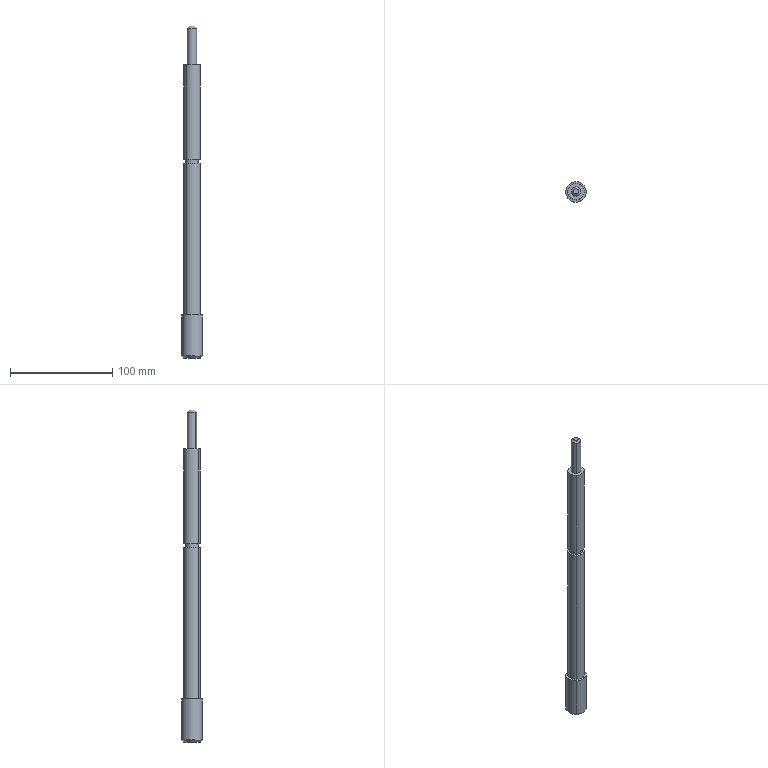Component | SolidWorks | 12-1 | 1 solid | 26 faces | box 20 x 20 x 324 mm | volume 64045 mm3 | cylinder 13 | plane 9 | cone 4 | commonest cylinder face diameters 16 x4 5 x3 9 x2 12 x2 20 x2
build123d program:
from build123d import *

# Parameters (mm, degrees)
CHAMFER1_SIZE      = 2
CUT_EXTRUDE1_START = -8
CUT_EXTRUDE1_DEPTH = 1.8


with BuildPart() as part:
    # Sketch1 → Revolve1 (revolve)
    with BuildSketch(Plane.XY, mode=Mode.PRIVATE) as revolve1_sk:
        Polygon((0, 0), (0, 10), (42, 10), (42, 8), (190, 8), (190, 6), (194, 6), (194, 8), (286, 8), (286, 4.5), (324, 4.5), (324, 0), align=None)
    revolve(revolve1_sk.sketch.rotate(Axis((324, 0, 0), (-1, 0, 0)), 90), axis=Axis((324, 0, 0), (-1, 0, 0)))

    # Chamfer1
    chamfer1_edges = [part.edges().sort_by_distance(p)[0] for p in [
        (0, 0, 10),
        (324, 0, 4.5),
    ]]
    chamfer(chamfer1_edges, length=CHAMFER1_SIZE)

    # Sketch2 → Cut-Extrude1 (cut)
    with BuildSketch(Plane.XY.offset(CUT_EXTRUDE1_START)):
        with BuildLine():
            Line((107, 2.5), (116, 2.5))
            ThreePointArc((116, 2.5), (118.5, 0), (116, -2.5))
            Line((116, -2.5), (107, -2.5))
            ThreePointArc((107, -2.5), (104.5, 0), (107, 2.5))
        make_face()
    extrude(amount=CUT_EXTRUDE1_DEPTH, mode=Mode.SUBTRACT)


solid = part.part

# Placed as in the assembly
solid = solid.moved(Location((-135.043, 380.991, 493.213), (90, -40.335, 90)))
STEP:
#1=COLOUR_RGB('',0.7922,0.8196,0.9333);
#2=FILL_AREA_STYLE_COLOUR('',#1);
#3=FILL_AREA_STYLE('',(#2));
#4=SURFACE_STYLE_FILL_AREA(#3);
#5=SURFACE_SIDE_STYLE('',(#4));
#6=SURFACE_STYLE_USAGE(.BOTH.,#5);
#7=PRESENTATION_STYLE_ASSIGNMENT((#6));
#8=CARTESIAN_POINT('',(-5.234,15.249,23.63));
#9=VERTEX_POINT('',#8);
#10=CARTESIAN_POINT('',(-5.159,15.186,23.532));
#11=VERTEX_POINT('',#10);
#12=CARTESIAN_POINT('',(-5.159,15.186,23.63));
#13=DIRECTION('',(-0.6473,-0.7623,0.));
#14=DIRECTION('',(0.,0.,1.));
#15=AXIS2_PLACEMENT_3D('',#12,#13,#14);
#16=CIRCLE('',#15,0.09843);
#17=EDGE_CURVE('',#9,#11,#16,.T.);
#18=ORIENTED_EDGE('',*,*,#17,.T.);
#19=CARTESIAN_POINT('',(-5.113,15.24,23.532));
#20=VERTEX_POINT('',#19);
#21=CARTESIAN_POINT('',(-5.159,15.186,23.532));
#22=DIRECTION('',(0.6473,0.7623,-0.));
#23=VECTOR('',#22,39.37);
#24=LINE('',#21,#23);
#25=EDGE_CURVE('',#11,#20,#24,.T.);
#26=ORIENTED_EDGE('',*,*,#25,.T.);
#27=CARTESIAN_POINT('',(-5.198,15.291,23.63));
#28=VERTEX_POINT('',#27);
#29=CARTESIAN_POINT('',(-5.198,15.291,23.63));
#30=CARTESIAN_POINT('',(-5.198,15.291,23.624));
#31=CARTESIAN_POINT('',(-5.197,15.291,23.617));
#32=CARTESIAN_POINT('',(-5.195,15.29,23.605));
#33=CARTESIAN_POINT('',(-5.193,15.289,23.599));
#34=CARTESIAN_POINT('',(-5.188,15.287,23.587));
#35=CARTESIAN_POINT('',(-5.185,15.286,23.581));
#36=CARTESIAN_POINT('',(-5.179,15.283,23.57));
#37=CARTESIAN_POINT('',(-5.175,15.281,23.565));
#38=CARTESIAN_POINT('',(-5.163,15.275,23.552));
#39=CARTESIAN_POINT('',(-5.153,15.269,23.544));
#40=CARTESIAN_POINT('',(-5.138,15.259,23.537));
#41=CARTESIAN_POINT('',(-5.133,15.256,23.535));
#42=CARTESIAN_POINT('',(-5.123,15.248,23.533));
#43=CARTESIAN_POINT('',(-5.118,15.244,23.532));
#44=CARTESIAN_POINT('',(-5.113,15.24,23.532));
#45=B_SPLINE_CURVE_WITH_KNOTS('',3,(#29,#30,#31,#32,#33,#34,#35,#36,#37,#38,#39,#40,#41,#42,#43,#44),.UNSPECIFIED.,.F.,.F.,(4,2,2,2,2,2,2,4),(0.,0.0004917,0.0009835,0.001475,0.001967,0.00295,0.003442,0.003934),.UNSPECIFIED.);
#46=EDGE_CURVE('',#28,#20,#45,.T.);
#47=ORIENTED_EDGE('',*,*,#46,.F.);
#48=CARTESIAN_POINT('',(-5.234,15.249,23.63));
#49=DIRECTION('',(0.6473,0.7623,-0.));
#50=VECTOR('',#49,39.37);
#51=LINE('',#48,#50);
#52=EDGE_CURVE('',#9,#28,#51,.T.);
#53=ORIENTED_EDGE('',*,*,#52,.F.);
#54=EDGE_LOOP('',(#18,#26,#47,#53));
#55=FACE_OUTER_BOUND('',#54,.T.);
#56=CARTESIAN_POINT('',(-5.159,15.186,23.63));
#57=DIRECTION('',(0.6473,0.7623,-0.));
#58=DIRECTION('',(0.,0.,-1.));
#59=AXIS2_PLACEMENT_3D('',#56,#57,#58);
#60=CYLINDRICAL_SURFACE('',#59,0.09843);
#61=ADVANCED_FACE('',(#55),#60,.F.);
#62=CARTESIAN_POINT('',(-5.521,14.76,19.418));
#63=VERTEX_POINT('',#62);
#64=CARTESIAN_POINT('',(-5.113,15.24,19.418));
#65=VERTEX_POINT('',#64);
#66=CARTESIAN_POINT('',(-5.317,15.,19.418));
#67=DIRECTION('',(-0.,-0.,-1.));
#68=DIRECTION('',(-0.6473,-0.7623,0.));
#69=AXIS2_PLACEMENT_3D('',#66,#67,#68);
#70=CIRCLE('',#69,0.315);
#71=EDGE_CURVE('',#63,#65,#70,.T.);
#72=ORIENTED_EDGE('',*,*,#71,.F.);
#73=CARTESIAN_POINT('',(-5.571,14.7,19.497));
#74=VERTEX_POINT('',#73);
#75=CARTESIAN_POINT('',(-5.571,14.7,19.497));
#76=DIRECTION('',(-0.4577,-0.539,0.7071));
#77=VECTOR('',#76,39.37);
#78=LINE('',#75,#77);
#79=EDGE_CURVE('',#63,#74,#78,.T.);
#80=ORIENTED_EDGE('',*,*,#79,.T.);
#81=CARTESIAN_POINT('',(-5.062,15.3,19.497));
#82=VERTEX_POINT('',#81);
#83=CARTESIAN_POINT('',(-5.317,15.,19.497));
#84=DIRECTION('',(0.,0.,1.));
#85=DIRECTION('',(-0.6473,-0.7623,0.));
#86=AXIS2_PLACEMENT_3D('',#83,#84,#85);
#87=CIRCLE('',#86,0.3937);
#88=EDGE_CURVE('',#82,#74,#87,.T.);
#89=ORIENTED_EDGE('',*,*,#88,.F.);
#90=CARTESIAN_POINT('',(-5.062,15.3,19.497));
#91=DIRECTION('',(0.4577,0.539,0.7071));
#92=VECTOR('',#91,39.37);
#93=LINE('',#90,#92);
#94=EDGE_CURVE('',#65,#82,#93,.T.);
#95=ORIENTED_EDGE('',*,*,#94,.F.);
#96=EDGE_LOOP('',(#72,#80,#89,#95));
#97=FACE_OUTER_BOUND('',#96,.T.);
#98=CARTESIAN_POINT('',(-5.317,15.,19.497));
#99=DIRECTION('',(0.,0.,1.));
#100=DIRECTION('',(0.6473,0.7623,0.));
#101=AXIS2_PLACEMENT_3D('',#98,#99,#100);
#102=CONICAL_SURFACE('',#101,0.3937,0.7854);
#103=ADVANCED_FACE('',(#97),#102,.T.);
#104=CARTESIAN_POINT('',(-5.253,15.075,32.174));
#105=VERTEX_POINT('',#104);
#106=CARTESIAN_POINT('',(-5.38,14.925,32.174));
#107=VERTEX_POINT('',#106);
#108=CARTESIAN_POINT('',(-5.317,15.,32.174));
#109=DIRECTION('',(0.,0.,1.));
#110=DIRECTION('',(0.6473,0.7623,0.));
#111=AXIS2_PLACEMENT_3D('',#108,#109,#110);
#112=CIRCLE('',#111,0.09843);
#113=EDGE_CURVE('',#105,#107,#112,.T.);
#114=ORIENTED_EDGE('',*,*,#113,.F.);
#115=CARTESIAN_POINT('',(-5.202,15.135,32.095));
#116=VERTEX_POINT('',#115);
#117=CARTESIAN_POINT('',(-5.253,15.075,32.174));
#118=DIRECTION('',(0.4577,0.539,-0.7071));
#119=VECTOR('',#118,39.37);
#120=LINE('',#117,#119);
#121=EDGE_CURVE('',#105,#116,#120,.T.);
#122=ORIENTED_EDGE('',*,*,#121,.T.);
#123=CARTESIAN_POINT('',(-5.431,14.865,32.095));
#124=VERTEX_POINT('',#123);
#125=CARTESIAN_POINT('',(-5.317,15.,32.095));
#126=DIRECTION('',(-0.,-0.,-1.));
#127=DIRECTION('',(0.6473,0.7623,0.));
#128=AXIS2_PLACEMENT_3D('',#125,#126,#127);
#129=CIRCLE('',#128,0.1772);
#130=EDGE_CURVE('',#124,#116,#129,.T.);
#131=ORIENTED_EDGE('',*,*,#130,.F.);
#132=CARTESIAN_POINT('',(-5.38,14.925,32.174));
#133=DIRECTION('',(-0.4577,-0.539,-0.7071));
#134=VECTOR('',#133,39.37);
#135=LINE('',#132,#134);
#136=EDGE_CURVE('',#107,#124,#135,.T.);
#137=ORIENTED_EDGE('',*,*,#136,.F.);
#138=EDGE_LOOP('',(#114,#122,#131,#137));
#139=FACE_OUTER_BOUND('',#138,.T.);
#140=CARTESIAN_POINT('',(-5.317,15.,32.174));
#141=DIRECTION('',(-0.,-0.,-1.));
#142=DIRECTION('',(-0.6473,-0.7623,0.));
#143=AXIS2_PLACEMENT_3D('',#140,#141,#142);
#144=CONICAL_SURFACE('',#143,0.09843,0.7854);
#145=ADVANCED_FACE('',(#139),#144,.T.);
#146=CARTESIAN_POINT('',(-5.202,15.135,30.678));
#147=VERTEX_POINT('',#146);
#148=CARTESIAN_POINT('',(-5.431,14.865,30.678));
#149=VERTEX_POINT('',#148);
#150=CARTESIAN_POINT('',(-5.317,15.,30.678));
#151=DIRECTION('',(0.,0.,1.));
#152=DIRECTION('',(0.6473,0.7623,0.));
#153=AXIS2_PLACEMENT_3D('',#150,#151,#152);
#154=CIRCLE('',#153,0.1772);
#155=EDGE_CURVE('',#147,#149,#154,.T.);
#156=ORIENTED_EDGE('',*,*,#155,.T.);
#157=CARTESIAN_POINT('',(-5.431,14.865,32.174));
#158=DIRECTION('',(0.,0.,1.));
#159=VECTOR('',#158,39.37);
#160=LINE('',#157,#159);
#161=EDGE_CURVE('',#149,#124,#160,.T.);
#162=ORIENTED_EDGE('',*,*,#161,.T.);
#163=ORIENTED_EDGE('',*,*,#130,.T.);
#164=CARTESIAN_POINT('',(-5.202,15.135,32.174));
#165=DIRECTION('',(0.,0.,1.));
#166=VECTOR('',#165,39.37);
#167=LINE('',#164,#166);
#168=EDGE_CURVE('',#147,#116,#167,.T.);
#169=ORIENTED_EDGE('',*,*,#168,.F.);
#170=EDGE_LOOP('',(#156,#162,#163,#169));
#171=FACE_OUTER_BOUND('',#170,.T.);
#172=CARTESIAN_POINT('',(-5.317,15.,32.174));
#173=DIRECTION('',(0.,0.,1.));
#174=DIRECTION('',(0.6473,0.7623,0.));
#175=AXIS2_PLACEMENT_3D('',#172,#173,#174);
#176=CYLINDRICAL_SURFACE('',#175,0.1772);
#177=ADVANCED_FACE('',(#171),#176,.T.);
#178=CARTESIAN_POINT('',(-5.113,15.24,27.056));
#179=VERTEX_POINT('',#178);
#180=CARTESIAN_POINT('',(-5.521,14.76,27.056));
#181=VERTEX_POINT('',#180);
#182=CARTESIAN_POINT('',(-5.317,15.,27.056));
#183=DIRECTION('',(0.,0.,1.));
#184=DIRECTION('',(0.6473,0.7623,0.));
#185=AXIS2_PLACEMENT_3D('',#182,#183,#184);
#186=CIRCLE('',#185,0.315);
#187=EDGE_CURVE('',#179,#181,#186,.T.);
#188=ORIENTED_EDGE('',*,*,#187,.T.);
#189=CARTESIAN_POINT('',(-5.521,14.76,30.678));
#190=VERTEX_POINT('',#189);
#191=CARTESIAN_POINT('',(-5.521,14.76,32.174));
#192=DIRECTION('',(0.,0.,1.));
#193=VECTOR('',#192,39.37);
#194=LINE('',#191,#193);
#195=EDGE_CURVE('',#181,#190,#194,.T.);
#196=ORIENTED_EDGE('',*,*,#195,.T.);
#197=CARTESIAN_POINT('',(-5.113,15.24,30.678));
#198=VERTEX_POINT('',#197);
#199=CARTESIAN_POINT('',(-5.317,15.,30.678));
#200=DIRECTION('',(0.,0.,1.));
#201=DIRECTION('',(0.6473,0.7623,0.));
#202=AXIS2_PLACEMENT_3D('',#199,#200,#201);
#203=CIRCLE('',#202,0.315);
#204=EDGE_CURVE('',#198,#190,#203,.T.);
#205=ORIENTED_EDGE('',*,*,#204,.F.);
#206=CARTESIAN_POINT('',(-5.113,15.24,32.174));
#207=DIRECTION('',(0.,0.,1.));
#208=VECTOR('',#207,39.37);
#209=LINE('',#206,#208);
#210=EDGE_CURVE('',#179,#198,#209,.T.);
#211=ORIENTED_EDGE('',*,*,#210,.F.);
#212=EDGE_LOOP('',(#188,#196,#205,#211));
#213=FACE_OUTER_BOUND('',#212,.T.);
#214=CARTESIAN_POINT('',(-5.317,15.,32.174));
#215=DIRECTION('',(0.,0.,1.));
#216=DIRECTION('',(0.6473,0.7623,0.));
#217=AXIS2_PLACEMENT_3D('',#214,#215,#216);
#218=CYLINDRICAL_SURFACE('',#217,0.315);
#219=ADVANCED_FACE('',(#213),#218,.T.);
#220=CARTESIAN_POINT('',(-5.164,15.18,26.898));
#221=VERTEX_POINT('',#220);
#222=CARTESIAN_POINT('',(-5.47,14.82,26.898));
#223=VERTEX_POINT('',#222);
#224=CARTESIAN_POINT('',(-5.317,15.,26.898));
#225=DIRECTION('',(0.,0.,1.));
#226=DIRECTION('',(0.6473,0.7623,0.));
#227=AXIS2_PLACEMENT_3D('',#224,#225,#226);
#228=CIRCLE('',#227,0.2362);
#229=EDGE_CURVE('',#221,#223,#228,.T.);
#230=ORIENTED_EDGE('',*,*,#229,.T.);
#231=CARTESIAN_POINT('',(-5.47,14.82,27.056));
#232=VERTEX_POINT('',#231);
#233=CARTESIAN_POINT('',(-5.47,14.82,32.174));
#234=DIRECTION('',(0.,0.,1.));
#235=VECTOR('',#234,39.37);
#236=LINE('',#233,#235);
#237=EDGE_CURVE('',#223,#232,#236,.T.);
#238=ORIENTED_EDGE('',*,*,#237,.T.);
#239=CARTESIAN_POINT('',(-5.164,15.18,27.056));
#240=VERTEX_POINT('',#239);
#241=CARTESIAN_POINT('',(-5.317,15.,27.056));
#242=DIRECTION('',(0.,0.,1.));
#243=DIRECTION('',(0.6473,0.7623,0.));
#244=AXIS2_PLACEMENT_3D('',#241,#242,#243);
#245=CIRCLE('',#244,0.2362);
#246=EDGE_CURVE('',#240,#232,#245,.T.);
#247=ORIENTED_EDGE('',*,*,#246,.F.);
#248=CARTESIAN_POINT('',(-5.164,15.18,32.174));
#249=DIRECTION('',(0.,0.,1.));
#250=VECTOR('',#249,39.37);
#251=LINE('',#248,#250);
#252=EDGE_CURVE('',#221,#240,#251,.T.);
#253=ORIENTED_EDGE('',*,*,#252,.F.);
#254=EDGE_LOOP('',(#230,#238,#247,#253));
#255=FACE_OUTER_BOUND('',#254,.T.);
#256=CARTESIAN_POINT('',(-5.317,15.,32.174));
#257=DIRECTION('',(0.,0.,1.));
#258=DIRECTION('',(0.6473,0.7623,0.));
#259=AXIS2_PLACEMENT_3D('',#256,#257,#258);
#260=CYLINDRICAL_SURFACE('',#259,0.2362);
#261=ADVANCED_FACE('',(#255),#260,.T.);
#262=ORIENTED_EDGE('',*,*,#88,.T.);
#263=CARTESIAN_POINT('',(-5.571,14.7,21.071));
#264=VERTEX_POINT('',#263);
#265=CARTESIAN_POINT('',(-5.571,14.7,32.174));
#266=DIRECTION('',(0.,0.,1.));
#267=VECTOR('',#266,39.37);
#268=LINE('',#265,#267);
#269=EDGE_CURVE('',#74,#264,#268,.T.);
#270=ORIENTED_EDGE('',*,*,#269,.T.);
#271=CARTESIAN_POINT('',(-5.062,15.3,21.071));
#272=VERTEX_POINT('',#271);
#273=CARTESIAN_POINT('',(-5.317,15.,21.071));
#274=DIRECTION('',(0.,0.,1.));
#275=DIRECTION('',(0.6473,0.7623,0.));
#276=AXIS2_PLACEMENT_3D('',#273,#274,#275);
#277=CIRCLE('',#276,0.3937);
#278=EDGE_CURVE('',#272,#264,#277,.T.);
#279=ORIENTED_EDGE('',*,*,#278,.F.);
#280=CARTESIAN_POINT('',(-5.062,15.3,32.174));
#281=DIRECTION('',(0.,0.,1.));
#282=VECTOR('',#281,39.37);
#283=LINE('',#280,#282);
#284=EDGE_CURVE('',#82,#272,#283,.T.);
#285=ORIENTED_EDGE('',*,*,#284,.F.);
#286=EDGE_LOOP('',(#262,#270,#279,#285));
#287=FACE_OUTER_BOUND('',#286,.T.);
#288=CARTESIAN_POINT('',(-5.317,15.,32.174));
#289=DIRECTION('',(0.,0.,1.));
#290=DIRECTION('',(0.6473,0.7623,0.));
#291=AXIS2_PLACEMENT_3D('',#288,#289,#290);
#292=CYLINDRICAL_SURFACE('',#291,0.3937);
#293=ADVANCED_FACE('',(#287),#292,.T.);
#294=CARTESIAN_POINT('',(-5.113,15.24,21.071));
#295=VERTEX_POINT('',#294);
#296=CARTESIAN_POINT('',(-5.521,14.76,21.071));
#297=VERTEX_POINT('',#296);
#298=CARTESIAN_POINT('',(-5.317,15.,21.071));
#299=DIRECTION('',(0.,0.,1.));
#300=DIRECTION('',(0.6473,0.7623,0.));
#301=AXIS2_PLACEMENT_3D('',#298,#299,#300);
#302=CIRCLE('',#301,0.315);
#303=EDGE_CURVE('',#295,#297,#302,.T.);
#304=ORIENTED_EDGE('',*,*,#303,.T.);
#305=CARTESIAN_POINT('',(-5.521,14.76,26.898));
#306=VERTEX_POINT('',#305);
#307=CARTESIAN_POINT('',(-5.521,14.76,32.174));
#308=DIRECTION('',(0.,0.,1.));
#309=VECTOR('',#308,39.37);
#310=LINE('',#307,#309);
#311=EDGE_CURVE('',#297,#306,#310,.T.);
#312=ORIENTED_EDGE('',*,*,#311,.T.);
#313=CARTESIAN_POINT('',(-5.113,15.24,26.898));
#314=VERTEX_POINT('',#313);
#315=CARTESIAN_POINT('',(-5.317,15.,26.898));
#316=DIRECTION('',(0.,0.,1.));
#317=DIRECTION('',(0.6473,0.7623,0.));
#318=AXIS2_PLACEMENT_3D('',#315,#316,#317);
#319=CIRCLE('',#318,0.315);
#320=EDGE_CURVE('',#314,#306,#319,.T.);
#321=ORIENTED_EDGE('',*,*,#320,.F.);
#322=CARTESIAN_POINT('',(-5.113,15.24,24.083));
#323=VERTEX_POINT('',#322);
#324=CARTESIAN_POINT('',(-5.113,15.24,32.174));
#325=DIRECTION('',(0.,0.,1.));
#326=VECTOR('',#325,39.37);
#327=LINE('',#324,#326);
#328=EDGE_CURVE('',#323,#314,#327,.T.);
#329=ORIENTED_EDGE('',*,*,#328,.F.);
#330=CARTESIAN_POINT('',(-5.198,15.291,23.985));
#331=VERTEX_POINT('',#330);
#332=CARTESIAN_POINT('',(-5.113,15.24,24.083));
#333=CARTESIAN_POINT('',(-5.118,15.244,24.083));
#334=CARTESIAN_POINT('',(-5.123,15.248,24.083));
#335=CARTESIAN_POINT('',(-5.133,15.256,24.08));
#336=CARTESIAN_POINT('',(-5.138,15.259,24.078));
#337=CARTESIAN_POINT('',(-5.148,15.266,24.073));
#338=CARTESIAN_POINT('',(-5.153,15.269,24.07));
#339=CARTESIAN_POINT('',(-5.162,15.274,24.063));
#340=CARTESIAN_POINT('',(-5.167,15.277,24.059));
#341=CARTESIAN_POINT('',(-5.175,15.281,24.05));
#342=CARTESIAN_POINT('',(-5.179,15.283,24.045));
#343=CARTESIAN_POINT('',(-5.185,15.286,24.034));
#344=CARTESIAN_POINT('',(-5.188,15.287,24.029));
#345=CARTESIAN_POINT('',(-5.193,15.289,24.017));
#346=CARTESIAN_POINT('',(-5.195,15.29,24.011));
#347=CARTESIAN_POINT('',(-5.197,15.291,23.998));
#348=CARTESIAN_POINT('',(-5.198,15.291,23.991));
#349=CARTESIAN_POINT('',(-5.198,15.291,23.985));
#350=B_SPLINE_CURVE_WITH_KNOTS('',3,(#332,#333,#334,#335,#336,#337,#338,#339,#340,#341,#342,#343,#344,#345,#346,#347,#348,#349),.UNSPECIFIED.,.F.,.F.,(4,2,2,2,2,2,2,2,4),(0.003934,0.004425,0.004916,0.005407,0.005898,0.006389,0.006881,0.007372,0.007863),.UNSPECIFIED.);
#351=EDGE_CURVE('',#323,#331,#350,.T.);
#352=ORIENTED_EDGE('',*,*,#351,.T.);
#353=CARTESIAN_POINT('',(-5.198,15.291,32.174));
#354=DIRECTION('',(-0.,-0.,-1.));
#355=VECTOR('',#354,39.37);
#356=LINE('',#353,#355);
#357=EDGE_CURVE('',#331,#28,#356,.T.);
#358=ORIENTED_EDGE('',*,*,#357,.T.);
#359=ORIENTED_EDGE('',*,*,#46,.T.);
#360=CARTESIAN_POINT('',(-5.113,15.24,32.174));
#361=DIRECTION('',(0.,0.,1.));
#362=VECTOR('',#361,39.37);
#363=LINE('',#360,#362);
#364=EDGE_CURVE('',#295,#20,#363,.T.);
#365=ORIENTED_EDGE('',*,*,#364,.F.);
#366=EDGE_LOOP('',(#304,#312,#321,#329,#352,#358,#359,#365));
#367=FACE_OUTER_BOUND('',#366,.T.);
#368=CARTESIAN_POINT('',(-5.317,15.,32.174));
#369=DIRECTION('',(0.,0.,1.));
#370=DIRECTION('',(0.6473,0.7623,0.));
#371=AXIS2_PLACEMENT_3D('',#368,#369,#370);
#372=CYLINDRICAL_SURFACE('',#371,0.315);
#373=ADVANCED_FACE('',(#367),#372,.T.);
#374=ORIENTED_EDGE('',*,*,#311,.F.);
#375=CARTESIAN_POINT('',(-5.317,15.,21.071));
#376=DIRECTION('',(0.,0.,1.));
#377=DIRECTION('',(0.6473,0.7623,0.));
#378=AXIS2_PLACEMENT_3D('',#375,#376,#377);
#379=CIRCLE('',#378,0.315);
#380=EDGE_CURVE('',#297,#295,#379,.T.);
#381=ORIENTED_EDGE('',*,*,#380,.T.);
#382=ORIENTED_EDGE('',*,*,#364,.T.);
#383=CARTESIAN_POINT('',(-5.048,15.164,23.63));
#384=VERTEX_POINT('',#383);
#385=CARTESIAN_POINT('',(-5.113,15.24,23.532));
#386=CARTESIAN_POINT('',(-5.108,15.236,23.532));
#387=CARTESIAN_POINT('',(-5.103,15.231,23.533));
#388=CARTESIAN_POINT('',(-5.094,15.222,23.535));
#389=CARTESIAN_POINT('',(-5.09,15.218,23.537));
#390=CARTESIAN_POINT('',(-5.081,15.209,23.542));
#391=CARTESIAN_POINT('',(-5.078,15.205,23.545));
#392=CARTESIAN_POINT('',(-5.071,15.196,23.552));
#393=CARTESIAN_POINT('',(-5.068,15.192,23.556));
#394=CARTESIAN_POINT('',(-5.062,15.185,23.565));
#395=CARTESIAN_POINT('',(-5.06,15.182,23.57));
#396=CARTESIAN_POINT('',(-5.055,15.176,23.581));
#397=CARTESIAN_POINT('',(-5.054,15.173,23.587));
#398=CARTESIAN_POINT('',(-5.051,15.169,23.599));
#399=CARTESIAN_POINT('',(-5.05,15.167,23.605));
#400=CARTESIAN_POINT('',(-5.048,15.165,23.617));
#401=CARTESIAN_POINT('',(-5.048,15.164,23.624));
#402=CARTESIAN_POINT('',(-5.048,15.164,23.63));
#403=B_SPLINE_CURVE_WITH_KNOTS('',3,(#385,#386,#387,#388,#389,#390,#391,#392,#393,#394,#395,#396,#397,#398,#399,#400,#401,#402),.UNSPECIFIED.,.F.,.F.,(4,2,2,2,2,2,2,2,4),(0.003934,0.004425,0.004916,0.005407,0.005898,0.006389,0.006881,0.007372,0.007863),.UNSPECIFIED.);
#404=EDGE_CURVE('',#20,#384,#403,.T.);
#405=ORIENTED_EDGE('',*,*,#404,.T.);
#406=CARTESIAN_POINT('',(-5.048,15.164,23.985));
#407=VERTEX_POINT('',#406);
#408=CARTESIAN_POINT('',(-5.048,15.164,32.174));
#409=DIRECTION('',(0.,0.,1.));
#410=VECTOR('',#409,39.37);
#411=LINE('',#408,#410);
#412=EDGE_CURVE('',#384,#407,#411,.T.);
#413=ORIENTED_EDGE('',*,*,#412,.T.);
#414=CARTESIAN_POINT('',(-5.048,15.164,23.985));
#415=CARTESIAN_POINT('',(-5.048,15.164,23.991));
#416=CARTESIAN_POINT('',(-5.048,15.165,23.998));
#417=CARTESIAN_POINT('',(-5.05,15.167,24.01));
#418=CARTESIAN_POINT('',(-5.051,15.169,24.017));
#419=CARTESIAN_POINT('',(-5.054,15.173,24.029));
#420=CARTESIAN_POINT('',(-5.055,15.176,24.034));
#421=CARTESIAN_POINT('',(-5.06,15.182,24.045));
#422=CARTESIAN_POINT('',(-5.062,15.185,24.05));
#423=CARTESIAN_POINT('',(-5.07,15.196,24.063));
#424=CARTESIAN_POINT('',(-5.077,15.205,24.071));
#425=CARTESIAN_POINT('',(-5.089,15.218,24.078));
#426=CARTESIAN_POINT('',(-5.094,15.222,24.08));
#427=CARTESIAN_POINT('',(-5.103,15.231,24.083));
#428=CARTESIAN_POINT('',(-5.108,15.236,24.083));
#429=CARTESIAN_POINT('',(-5.113,15.24,24.083));
#430=B_SPLINE_CURVE_WITH_KNOTS('',3,(#414,#415,#416,#417,#418,#419,#420,#421,#422,#423,#424,#425,#426,#427,#428,#429),.UNSPECIFIED.,.F.,.F.,(4,2,2,2,2,2,2,4),(0.,0.0004917,0.0009835,0.001475,0.001967,0.00295,0.003442,0.003934),.UNSPECIFIED.);
#431=EDGE_CURVE('',#407,#323,#430,.T.);
#432=ORIENTED_EDGE('',*,*,#431,.T.);
#433=ORIENTED_EDGE('',*,*,#328,.T.);
#434=CARTESIAN_POINT('',(-5.317,15.,26.898));
#435=DIRECTION('',(0.,0.,1.));
#436=DIRECTION('',(0.6473,0.7623,0.));
#437=AXIS2_PLACEMENT_3D('',#434,#435,#436);
#438=CIRCLE('',#437,0.315);
#439=EDGE_CURVE('',#306,#314,#438,.T.);
#440=ORIENTED_EDGE('',*,*,#439,.F.);
#441=EDGE_LOOP('',(#374,#381,#382,#405,#413,#432,#433,#440));
#442=FACE_OUTER_BOUND('',#441,.T.);
#443=CARTESIAN_POINT('',(-5.317,15.,32.174));
#444=DIRECTION('',(0.,0.,1.));
#445=DIRECTION('',(0.6473,0.7623,0.));
#446=AXIS2_PLACEMENT_3D('',#443,#444,#445);
#447=CYLINDRICAL_SURFACE('',#446,0.315);
#448=ADVANCED_FACE('',(#442),#447,.T.);
#449=CARTESIAN_POINT('',(-5.317,15.,19.418));
#450=DIRECTION('',(-0.,-0.,-1.));
#451=DIRECTION('',(-0.6473,-0.7623,0.));
#452=AXIS2_PLACEMENT_3D('',#449,#450,#451);
#453=CIRCLE('',#452,0.315);
#454=EDGE_CURVE('',#65,#63,#453,.T.);
#455=ORIENTED_EDGE('',*,*,#454,.T.);
#456=ORIENTED_EDGE('',*,*,#71,.T.);
#457=EDGE_LOOP('',(#455,#456));
#458=FACE_OUTER_BOUND('',#457,.T.);
#459=CARTESIAN_POINT('',(-5.317,15.,19.418));
#460=DIRECTION('',(-0.,-0.,-1.));
#461=DIRECTION('',(-0.6473,-0.7623,0.));
#462=AXIS2_PLACEMENT_3D('',#459,#460,#461);
#463=PLANE('',#462);
#464=ADVANCED_FACE('',(#458),#463,.T.);
#465=ORIENTED_EDGE('',*,*,#269,.F.);
#466=CARTESIAN_POINT('',(-5.317,15.,19.497));
#467=DIRECTION('',(0.,0.,1.));
#468=DIRECTION('',(-0.6473,-0.7623,0.));
#469=AXIS2_PLACEMENT_3D('',#466,#467,#468);
#470=CIRCLE('',#469,0.3937);
#471=EDGE_CURVE('',#74,#82,#470,.T.);
#472=ORIENTED_EDGE('',*,*,#471,.T.);
#473=ORIENTED_EDGE('',*,*,#284,.T.);
#474=CARTESIAN_POINT('',(-5.317,15.,21.071));
#475=DIRECTION('',(0.,0.,1.));
#476=DIRECTION('',(0.6473,0.7623,0.));
#477=AXIS2_PLACEMENT_3D('',#474,#475,#476);
#478=CIRCLE('',#477,0.3937);
#479=EDGE_CURVE('',#264,#272,#478,.T.);
#480=ORIENTED_EDGE('',*,*,#479,.F.);
#481=EDGE_LOOP('',(#465,#472,#473,#480));
#482=FACE_OUTER_BOUND('',#481,.T.);
#483=CARTESIAN_POINT('',(-5.317,15.,32.174));
#484=DIRECTION('',(0.,0.,1.));
#485=DIRECTION('',(0.6473,0.7623,0.));
#486=AXIS2_PLACEMENT_3D('',#483,#484,#485);
#487=CYLINDRICAL_SURFACE('',#486,0.3937);
#488=ADVANCED_FACE('',(#482),#487,.T.);
#489=ORIENTED_EDGE('',*,*,#278,.T.);
#490=ORIENTED_EDGE('',*,*,#479,.T.);
#491=EDGE_LOOP('',(#489,#490));
#492=FACE_OUTER_BOUND('',#491,.T.);
#493=ORIENTED_EDGE('',*,*,#303,.F.);
#494=ORIENTED_EDGE('',*,*,#380,.F.);
#495=EDGE_LOOP('',(#493,#494));
#496=FACE_BOUND('',#495,.T.);
#497=CARTESIAN_POINT('',(-5.617,15.254,21.071));
#498=DIRECTION('',(0.,0.,1.));
#499=DIRECTION('',(0.6473,0.7623,-0.));
#500=AXIS2_PLACEMENT_3D('',#497,#498,#499);
#501=PLANE('',#500);
#502=ADVANCED_FACE('',(#492,#496),#501,.T.);
#503=ORIENTED_EDGE('',*,*,#320,.T.);
#504=ORIENTED_EDGE('',*,*,#439,.T.);
#505=EDGE_LOOP('',(#503,#504));
#506=FACE_OUTER_BOUND('',#505,.T.);
#507=ORIENTED_EDGE('',*,*,#229,.F.);
#508=CARTESIAN_POINT('',(-5.317,15.,26.898));
#509=DIRECTION('',(0.,0.,1.));
#510=DIRECTION('',(0.6473,0.7623,0.));
#511=AXIS2_PLACEMENT_3D('',#508,#509,#510);
#512=CIRCLE('',#511,0.2362);
#513=EDGE_CURVE('',#223,#221,#512,.T.);
#514=ORIENTED_EDGE('',*,*,#513,.F.);
#515=EDGE_LOOP('',(#507,#514));
#516=FACE_BOUND('',#515,.T.);
#517=CARTESIAN_POINT('',(-5.557,15.204,26.898));
#518=DIRECTION('',(0.,0.,1.));
#519=DIRECTION('',(0.6473,0.7623,-0.));
#520=AXIS2_PLACEMENT_3D('',#517,#518,#519);
#521=PLANE('',#520);
#522=ADVANCED_FACE('',(#506,#516),#521,.T.);
#523=ORIENTED_EDGE('',*,*,#237,.F.);
#524=ORIENTED_EDGE('',*,*,#513,.T.);
#525=ORIENTED_EDGE('',*,*,#252,.T.);
#526=CARTESIAN_POINT('',(-5.317,15.,27.056));
#527=DIRECTION('',(0.,0.,1.));
#528=DIRECTION('',(0.6473,0.7623,0.));
#529=AXIS2_PLACEMENT_3D('',#526,#527,#528);
#530=CIRCLE('',#529,0.2362);
#531=EDGE_CURVE('',#232,#240,#530,.T.);
#532=ORIENTED_EDGE('',*,*,#531,.F.);
#533=EDGE_LOOP('',(#523,#524,#525,#532));
#534=FACE_OUTER_BOUND('',#533,.T.);
#535=CARTESIAN_POINT('',(-5.317,15.,32.174));
#536=DIRECTION('',(0.,0.,1.));
#537=DIRECTION('',(0.6473,0.7623,0.));
#538=AXIS2_PLACEMENT_3D('',#535,#536,#537);
#539=CYLINDRICAL_SURFACE('',#538,0.2362);
#540=ADVANCED_FACE('',(#534),#539,.T.);
#541=ORIENTED_EDGE('',*,*,#246,.T.);
#542=ORIENTED_EDGE('',*,*,#531,.T.);
#543=EDGE_LOOP('',(#541,#542));
#544=FACE_BOUND('',#543,.T.);
#545=ORIENTED_EDGE('',*,*,#187,.F.);
#546=CARTESIAN_POINT('',(-5.317,15.,27.056));
#547=DIRECTION('',(0.,0.,1.));
#548=DIRECTION('',(0.6473,0.7623,0.));
#549=AXIS2_PLACEMENT_3D('',#546,#547,#548);
#550=CIRCLE('',#549,0.315);
#551=EDGE_CURVE('',#181,#179,#550,.T.);
#552=ORIENTED_EDGE('',*,*,#551,.F.);
#553=EDGE_LOOP('',(#545,#552));
#554=FACE_OUTER_BOUND('',#553,.T.);
#555=CARTESIAN_POINT('',(-5.497,15.153,27.056));
#556=DIRECTION('',(-0.,-0.,-1.));
#557=DIRECTION('',(-0.6473,-0.7623,0.));
#558=AXIS2_PLACEMENT_3D('',#555,#556,#557);
#559=PLANE('',#558);
#560=ADVANCED_FACE('',(#544,#554),#559,.T.);
#561=ORIENTED_EDGE('',*,*,#195,.F.);
#562=ORIENTED_EDGE('',*,*,#551,.T.);
#563=ORIENTED_EDGE('',*,*,#210,.T.);
#564=CARTESIAN_POINT('',(-5.317,15.,30.678));
#565=DIRECTION('',(0.,0.,1.));
#566=DIRECTION('',(0.6473,0.7623,0.));
#567=AXIS2_PLACEMENT_3D('',#564,#565,#566);
#568=CIRCLE('',#567,0.315);
#569=EDGE_CURVE('',#190,#198,#568,.T.);
#570=ORIENTED_EDGE('',*,*,#569,.F.);
#571=EDGE_LOOP('',(#561,#562,#563,#570));
#572=FACE_OUTER_BOUND('',#571,.T.);
#573=CARTESIAN_POINT('',(-5.317,15.,32.174));
#574=DIRECTION('',(0.,0.,1.));
#575=DIRECTION('',(0.6473,0.7623,0.));
#576=AXIS2_PLACEMENT_3D('',#573,#574,#575);
#577=CYLINDRICAL_SURFACE('',#576,0.315);
#578=ADVANCED_FACE('',(#572),#577,.T.);
#579=ORIENTED_EDGE('',*,*,#204,.T.);
#580=ORIENTED_EDGE('',*,*,#569,.T.);
#581=EDGE_LOOP('',(#579,#580));
#582=FACE_OUTER_BOUND('',#581,.T.);
#583=ORIENTED_EDGE('',*,*,#155,.F.);
#584=CARTESIAN_POINT('',(-5.317,15.,30.678));
#585=DIRECTION('',(0.,0.,1.));
#586=DIRECTION('',(0.6473,0.7623,0.));
#587=AXIS2_PLACEMENT_3D('',#584,#585,#586);
#588=CIRCLE('',#587,0.1772);
#589=EDGE_CURVE('',#149,#147,#588,.T.);
#590=ORIENTED_EDGE('',*,*,#589,.F.);
#591=EDGE_LOOP('',(#583,#590));
#592=FACE_BOUND('',#591,.T.);
#593=CARTESIAN_POINT('',(-5.557,15.204,30.678));
#594=DIRECTION('',(0.,0.,1.));
#595=DIRECTION('',(0.6473,0.7623,-0.));
#596=AXIS2_PLACEMENT_3D('',#593,#594,#595);
#597=PLANE('',#596);
#598=ADVANCED_FACE('',(#582,#592),#597,.T.);
#599=ORIENTED_EDGE('',*,*,#161,.F.);
#600=ORIENTED_EDGE('',*,*,#589,.T.);
#601=ORIENTED_EDGE('',*,*,#168,.T.);
#602=CARTESIAN_POINT('',(-5.317,15.,32.095));
#603=DIRECTION('',(-0.,-0.,-1.));
#604=DIRECTION('',(0.6473,0.7623,0.));
#605=AXIS2_PLACEMENT_3D('',#602,#603,#604);
#606=CIRCLE('',#605,0.1772);
#607=EDGE_CURVE('',#116,#124,#606,.T.);
#608=ORIENTED_EDGE('',*,*,#607,.T.);
#609=EDGE_LOOP('',(#599,#600,#601,#608));
#610=FACE_OUTER_BOUND('',#609,.T.);
#611=CARTESIAN_POINT('',(-5.317,15.,32.174));
#612=DIRECTION('',(0.,0.,1.));
#613=DIRECTION('',(0.6473,0.7623,0.));
#614=AXIS2_PLACEMENT_3D('',#611,#612,#613);
#615=CYLINDRICAL_SURFACE('',#614,0.1772);
#616=ADVANCED_FACE('',(#610),#615,.T.);
#617=CARTESIAN_POINT('',(-5.317,15.,32.174));
#618=DIRECTION('',(0.,0.,1.));
#619=DIRECTION('',(0.6473,0.7623,0.));
#620=AXIS2_PLACEMENT_3D('',#617,#618,#619);
#621=CIRCLE('',#620,0.09843);
#622=EDGE_CURVE('',#107,#105,#621,.T.);
#623=ORIENTED_EDGE('',*,*,#622,.T.);
#624=ORIENTED_EDGE('',*,*,#113,.T.);
#625=EDGE_LOOP('',(#623,#624));
#626=FACE_OUTER_BOUND('',#625,.T.);
#627=CARTESIAN_POINT('',(-5.452,15.114,32.174));
#628=DIRECTION('',(0.,0.,1.));
#629=DIRECTION('',(0.6473,0.7623,-0.));
#630=AXIS2_PLACEMENT_3D('',#627,#628,#629);
#631=PLANE('',#630);
#632=ADVANCED_FACE('',(#626),#631,.T.);
#633=ORIENTED_EDGE('',*,*,#121,.F.);
#634=ORIENTED_EDGE('',*,*,#622,.F.);
#635=ORIENTED_EDGE('',*,*,#136,.T.);
#636=ORIENTED_EDGE('',*,*,#607,.F.);
#637=EDGE_LOOP('',(#633,#634,#635,#636));
#638=FACE_OUTER_BOUND('',#637,.T.);
#639=CARTESIAN_POINT('',(-5.317,15.,32.174));
#640=DIRECTION('',(-0.,-0.,-1.));
#641=DIRECTION('',(-0.6473,-0.7623,0.));
#642=AXIS2_PLACEMENT_3D('',#639,#640,#641);
#643=CONICAL_SURFACE('',#642,0.09843,0.7854);
#644=ADVANCED_FACE('',(#638),#643,.T.);
#645=ORIENTED_EDGE('',*,*,#79,.F.);
#646=ORIENTED_EDGE('',*,*,#454,.F.);
#647=ORIENTED_EDGE('',*,*,#94,.T.);
#648=ORIENTED_EDGE('',*,*,#471,.F.);
#649=EDGE_LOOP('',(#645,#646,#647,#648));
#650=FACE_OUTER_BOUND('',#649,.T.);
#651=CARTESIAN_POINT('',(-5.317,15.,19.497));
#652=DIRECTION('',(0.,0.,1.));
#653=DIRECTION('',(0.6473,0.7623,0.));
#654=AXIS2_PLACEMENT_3D('',#651,#652,#653);
#655=CONICAL_SURFACE('',#654,0.3937,0.7854);
#656=ADVANCED_FACE('',(#650),#655,.T.);
#657=ORIENTED_EDGE('',*,*,#25,.F.);
#658=CARTESIAN_POINT('',(-5.084,15.122,23.63));
#659=VERTEX_POINT('',#658);
#660=CARTESIAN_POINT('',(-5.159,15.186,23.63));
#661=DIRECTION('',(-0.6473,-0.7623,0.));
#662=DIRECTION('',(0.,0.,1.));
#663=AXIS2_PLACEMENT_3D('',#660,#661,#662);
#664=CIRCLE('',#663,0.09843);
#665=EDGE_CURVE('',#11,#659,#664,.T.);
#666=ORIENTED_EDGE('',*,*,#665,.T.);
#667=CARTESIAN_POINT('',(-5.084,15.122,23.63));
#668=DIRECTION('',(0.6473,0.7623,-0.));
#669=VECTOR('',#668,39.37);
#670=LINE('',#667,#669);
#671=EDGE_CURVE('',#659,#384,#670,.T.);
#672=ORIENTED_EDGE('',*,*,#671,.T.);
#673=ORIENTED_EDGE('',*,*,#404,.F.);
#674=EDGE_LOOP('',(#657,#666,#672,#673));
#675=FACE_OUTER_BOUND('',#674,.T.);
#676=CARTESIAN_POINT('',(-5.159,15.186,23.63));
#677=DIRECTION('',(0.6473,0.7623,-0.));
#678=DIRECTION('',(0.,0.,-1.));
#679=AXIS2_PLACEMENT_3D('',#676,#677,#678);
#680=CYLINDRICAL_SURFACE('',#679,0.09843);
#681=ADVANCED_FACE('',(#675),#680,.F.);
#682=ORIENTED_EDGE('',*,*,#671,.F.);
#683=CARTESIAN_POINT('',(-5.084,15.122,23.985));
#684=VERTEX_POINT('',#683);
#685=CARTESIAN_POINT('',(-5.084,15.122,23.63));
#686=DIRECTION('',(0.,0.,1.));
#687=VECTOR('',#686,39.37);
#688=LINE('',#685,#687);
#689=EDGE_CURVE('',#659,#684,#688,.T.);
#690=ORIENTED_EDGE('',*,*,#689,.T.);
#691=CARTESIAN_POINT('',(-5.084,15.122,23.985));
#692=DIRECTION('',(0.6473,0.7623,-0.));
#693=VECTOR('',#692,39.37);
#694=LINE('',#691,#693);
#695=EDGE_CURVE('',#684,#407,#694,.T.);
#696=ORIENTED_EDGE('',*,*,#695,.T.);
#697=ORIENTED_EDGE('',*,*,#412,.F.);
#698=EDGE_LOOP('',(#682,#690,#696,#697));
#699=FACE_OUTER_BOUND('',#698,.T.);
#700=CARTESIAN_POINT('',(-5.084,15.122,23.63));
#701=DIRECTION('',(-0.7623,0.6473,-0.));
#702=DIRECTION('',(-0.6473,-0.7623,0.));
#703=AXIS2_PLACEMENT_3D('',#700,#701,#702);
#704=PLANE('',#703);
#705=ADVANCED_FACE('',(#699),#704,.T.);
#706=ORIENTED_EDGE('',*,*,#695,.F.);
#707=CARTESIAN_POINT('',(-5.234,15.249,23.985));
#708=VERTEX_POINT('',#707);
#709=CARTESIAN_POINT('',(-5.159,15.186,23.985));
#710=DIRECTION('',(-0.6473,-0.7623,0.));
#711=DIRECTION('',(0.,0.,1.));
#712=AXIS2_PLACEMENT_3D('',#709,#710,#711);
#713=CIRCLE('',#712,0.09843);
#714=EDGE_CURVE('',#684,#708,#713,.T.);
#715=ORIENTED_EDGE('',*,*,#714,.T.);
#716=CARTESIAN_POINT('',(-5.234,15.249,23.985));
#717=DIRECTION('',(0.6473,0.7623,-0.));
#718=VECTOR('',#717,39.37);
#719=LINE('',#716,#718);
#720=EDGE_CURVE('',#708,#331,#719,.T.);
#721=ORIENTED_EDGE('',*,*,#720,.T.);
#722=ORIENTED_EDGE('',*,*,#351,.F.);
#723=ORIENTED_EDGE('',*,*,#431,.F.);
#724=EDGE_LOOP('',(#706,#715,#721,#722,#723));
#725=FACE_OUTER_BOUND('',#724,.T.);
#726=CARTESIAN_POINT('',(-5.159,15.186,23.985));
#727=DIRECTION('',(0.6473,0.7623,-0.));
#728=DIRECTION('',(0.,0.,-1.));
#729=AXIS2_PLACEMENT_3D('',#726,#727,#728);
#730=CYLINDRICAL_SURFACE('',#729,0.09843);
#731=ADVANCED_FACE('',(#725),#730,.F.);
#732=ORIENTED_EDGE('',*,*,#720,.F.);
#733=CARTESIAN_POINT('',(-5.234,15.249,23.63));
#734=DIRECTION('',(-0.,-0.,-1.));
#735=VECTOR('',#734,39.37);
#736=LINE('',#733,#735);
#737=EDGE_CURVE('',#708,#9,#736,.T.);
#738=ORIENTED_EDGE('',*,*,#737,.T.);
#739=ORIENTED_EDGE('',*,*,#52,.T.);
#740=ORIENTED_EDGE('',*,*,#357,.F.);
#741=EDGE_LOOP('',(#732,#738,#739,#740));
#742=FACE_OUTER_BOUND('',#741,.T.);
#743=CARTESIAN_POINT('',(-5.234,15.249,23.63));
#744=DIRECTION('',(0.7623,-0.6473,0.));
#745=DIRECTION('',(0.6473,0.7623,-0.));
#746=AXIS2_PLACEMENT_3D('',#743,#744,#745);
#747=PLANE('',#746);
#748=ADVANCED_FACE('',(#742),#747,.T.);
#749=ORIENTED_EDGE('',*,*,#17,.F.);
#750=ORIENTED_EDGE('',*,*,#737,.F.);
#751=ORIENTED_EDGE('',*,*,#714,.F.);
#752=ORIENTED_EDGE('',*,*,#689,.F.);
#753=ORIENTED_EDGE('',*,*,#665,.F.);
#754=EDGE_LOOP('',(#749,#750,#751,#752,#753));
#755=FACE_OUTER_BOUND('',#754,.T.);
#756=CARTESIAN_POINT('',(-5.159,15.186,23.63));
#757=DIRECTION('',(-0.6473,-0.7623,0.));
#758=DIRECTION('',(0.,0.,1.));
#759=AXIS2_PLACEMENT_3D('',#756,#757,#758);
#760=PLANE('',#759);
#761=ADVANCED_FACE('',(#755),#760,.F.);
#762=CLOSED_SHELL('',(#61,#103,#145,#177,#219,#261,#293,#373,#448,#464,#488,#502,#522,#540,#560,#578,#598,#616,#632,#644,#656,#681,#705,#731,#748,#761));
#763=MANIFOLD_SOLID_BREP('',#762);
#764=STYLED_ITEM('',(#7),#763);
#765=PRESENTATION_LAYER_ASSIGNMENT('','',(#764));
#766=(LENGTH_UNIT()NAMED_UNIT(*)SI_UNIT($,.METRE.));
#767=LENGTH_MEASURE_WITH_UNIT(LENGTH_MEASURE(0.0254),#766);
#768=DIMENSIONAL_EXPONENTS(1.,0.,0.,0.,0.,0.,0.);
#769=(CONVERSION_BASED_UNIT('',#767)LENGTH_UNIT()NAMED_UNIT(#768));
#770=UNCERTAINTY_MEASURE_WITH_UNIT(LENGTH_MEASURE(0.00001),#769,'','');
#771=(NAMED_UNIT(*)PLANE_ANGLE_UNIT()SI_UNIT($,.RADIAN.));
#772=(NAMED_UNIT(*)SI_UNIT($,.STERADIAN.)SOLID_ANGLE_UNIT());
#773=(GEOMETRIC_REPRESENTATION_CONTEXT(3)GLOBAL_UNCERTAINTY_ASSIGNED_CONTEXT((#770))GLOBAL_UNIT_ASSIGNED_CONTEXT((#769,#771,#772))REPRESENTATION_CONTEXT('',''));
#774=MECHANICAL_DESIGN_GEOMETRIC_PRESENTATION_REPRESENTATION('',(#764),#773);
#775=CARTESIAN_POINT('',(0.,0.,0.));
#776=DIRECTION('',(0.,0.,1.));
#777=DIRECTION('',(1.,0.,0.));
#778=AXIS2_PLACEMENT_3D('',#775,#776,#777);
#779=(LENGTH_UNIT()NAMED_UNIT(*)SI_UNIT($,.METRE.));
#780=LENGTH_MEASURE_WITH_UNIT(LENGTH_MEASURE(0.0254),#779);
#781=DIMENSIONAL_EXPONENTS(1.,0.,0.,0.,0.,0.,0.);
#782=(CONVERSION_BASED_UNIT('',#780)LENGTH_UNIT()NAMED_UNIT(#781));
#783=UNCERTAINTY_MEASURE_WITH_UNIT(LENGTH_MEASURE(0.00001),#782,'','');
#784=(NAMED_UNIT(*)PLANE_ANGLE_UNIT()SI_UNIT($,.RADIAN.));
#785=(NAMED_UNIT(*)SI_UNIT($,.STERADIAN.)SOLID_ANGLE_UNIT());
#786=(GEOMETRIC_REPRESENTATION_CONTEXT(3)GLOBAL_UNCERTAINTY_ASSIGNED_CONTEXT((#783))GLOBAL_UNIT_ASSIGNED_CONTEXT((#782,#784,#785))REPRESENTATION_CONTEXT('',''));
#787=ADVANCED_BREP_SHAPE_REPRESENTATION('',(#763,#778),#786);